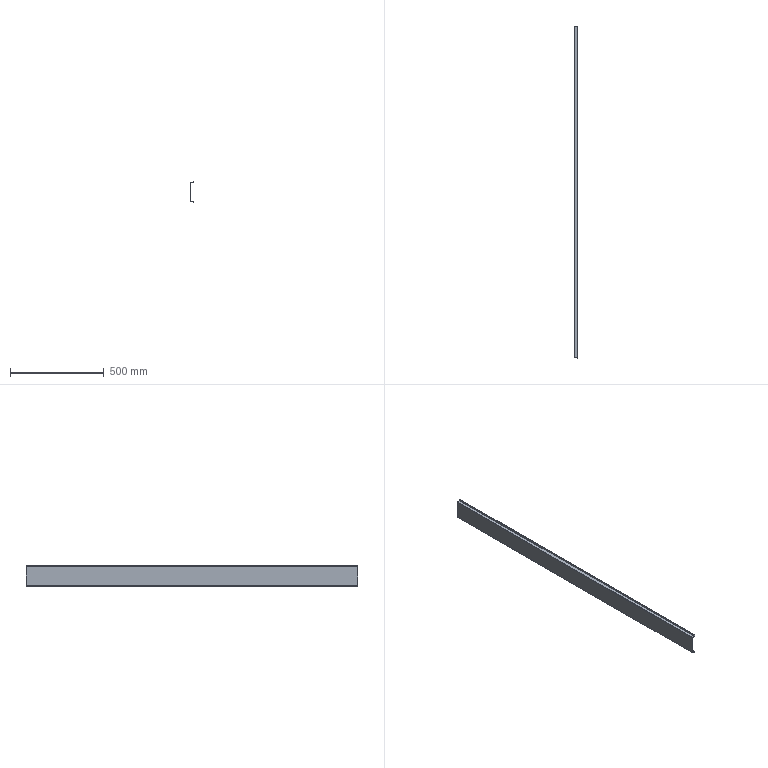Component | SolidWorks | RearDoorPanelWeldment-1_RearDoorStiffener-1 | 1 solid | 38 faces | box 18.9 x 1772 x 117 mm | volume 268936 mm3 | plane 30 | cylinder 8 | commonest cylinder face diameters 2.2 x4 0.2 x4
STEP:
#1=COLOUR_RGB('',0.7922,0.8196,0.9333);
#2=FILL_AREA_STYLE_COLOUR('',#1);
#3=FILL_AREA_STYLE('',(#2));
#4=SURFACE_STYLE_FILL_AREA(#3);
#5=SURFACE_SIDE_STYLE('',(#4));
#6=SURFACE_STYLE_USAGE(.BOTH.,#5);
#7=PRESENTATION_STYLE_ASSIGNMENT((#6));
#8=CARTESIAN_POINT('',(22.369,-36.828,72.855));
#9=VERTEX_POINT('',#8);
#10=CARTESIAN_POINT('',(23.027,-36.828,72.855));
#11=VERTEX_POINT('',#10);
#12=CARTESIAN_POINT('',(23.07,-36.828,72.855));
#13=DIRECTION('',(1.,0.,-0.));
#14=VECTOR('',#13,39.37);
#15=LINE('',#12,#14);
#16=EDGE_CURVE('',#9,#11,#15,.T.);
#17=ORIENTED_EDGE('',*,*,#16,.T.);
#18=CARTESIAN_POINT('',(23.027,-36.828,72.894));
#19=VERTEX_POINT('',#18);
#20=CARTESIAN_POINT('',(23.027,-36.828,72.855));
#21=DIRECTION('',(0.,0.,1.));
#22=VECTOR('',#21,39.37);
#23=LINE('',#20,#22);
#24=EDGE_CURVE('',#11,#19,#23,.T.);
#25=ORIENTED_EDGE('',*,*,#24,.T.);
#26=CARTESIAN_POINT('',(22.369,-36.828,72.894));
#27=VERTEX_POINT('',#26);
#28=CARTESIAN_POINT('',(22.326,-36.828,72.894));
#29=DIRECTION('',(1.,0.,-0.));
#30=VECTOR('',#29,39.37);
#31=LINE('',#28,#30);
#32=EDGE_CURVE('',#27,#19,#31,.T.);
#33=ORIENTED_EDGE('',*,*,#32,.F.);
#34=CARTESIAN_POINT('',(22.369,-36.828,72.855));
#35=DIRECTION('',(-0.,-0.,-1.));
#36=VECTOR('',#35,39.37);
#37=LINE('',#34,#36);
#38=EDGE_CURVE('',#27,#9,#37,.T.);
#39=ORIENTED_EDGE('',*,*,#38,.T.);
#40=EDGE_LOOP('',(#17,#25,#33,#39));
#41=FACE_OUTER_BOUND('',#40,.T.);
#42=CARTESIAN_POINT('',(23.07,-36.828,72.855));
#43=DIRECTION('',(0.,-1.,0.));
#44=DIRECTION('',(1.,0.,-0.));
#45=AXIS2_PLACEMENT_3D('',#42,#43,#44);
#46=PLANE('',#45);
#47=ADVANCED_FACE('',(#41),#46,.T.);
#48=CARTESIAN_POINT('',(23.027,32.936,72.855));
#49=VERTEX_POINT('',#48);
#50=CARTESIAN_POINT('',(22.369,32.936,72.855));
#51=VERTEX_POINT('',#50);
#52=CARTESIAN_POINT('',(22.365,32.936,72.855));
#53=DIRECTION('',(-1.,-0.,0.));
#54=VECTOR('',#53,39.37);
#55=LINE('',#52,#54);
#56=EDGE_CURVE('',#49,#51,#55,.T.);
#57=ORIENTED_EDGE('',*,*,#56,.F.);
#58=CARTESIAN_POINT('',(23.027,-36.828,72.855));
#59=DIRECTION('',(-0.,1.,-0.));
#60=VECTOR('',#59,39.37);
#61=LINE('',#58,#60);
#62=EDGE_CURVE('',#11,#49,#61,.T.);
#63=ORIENTED_EDGE('',*,*,#62,.F.);
#64=ORIENTED_EDGE('',*,*,#16,.F.);
#65=CARTESIAN_POINT('',(22.369,30.625,72.855));
#66=DIRECTION('',(-0.,1.,-0.));
#67=VECTOR('',#66,39.37);
#68=LINE('',#65,#67);
#69=EDGE_CURVE('',#9,#51,#68,.T.);
#70=ORIENTED_EDGE('',*,*,#69,.T.);
#71=EDGE_LOOP('',(#57,#63,#64,#70));
#72=FACE_OUTER_BOUND('',#71,.T.);
#73=CARTESIAN_POINT('',(22.326,30.625,72.855));
#74=DIRECTION('',(-0.,-0.,-1.));
#75=DIRECTION('',(1.,0.,-0.));
#76=AXIS2_PLACEMENT_3D('',#73,#74,#75);
#77=PLANE('',#76);
#78=ADVANCED_FACE('',(#72),#77,.T.);
#79=CARTESIAN_POINT('',(23.027,32.936,72.894));
#80=VERTEX_POINT('',#79);
#81=CARTESIAN_POINT('',(23.027,-36.828,72.894));
#82=DIRECTION('',(-0.,1.,-0.));
#83=VECTOR('',#82,39.37);
#84=LINE('',#81,#83);
#85=EDGE_CURVE('',#19,#80,#84,.T.);
#86=ORIENTED_EDGE('',*,*,#85,.T.);
#87=CARTESIAN_POINT('',(22.369,32.936,72.894));
#88=VERTEX_POINT('',#87);
#89=CARTESIAN_POINT('',(22.326,32.936,72.894));
#90=DIRECTION('',(-1.,-0.,0.));
#91=VECTOR('',#90,39.37);
#92=LINE('',#89,#91);
#93=EDGE_CURVE('',#80,#88,#92,.T.);
#94=ORIENTED_EDGE('',*,*,#93,.T.);
#95=CARTESIAN_POINT('',(22.369,-36.828,72.894));
#96=DIRECTION('',(-0.,1.,-0.));
#97=VECTOR('',#96,39.37);
#98=LINE('',#95,#97);
#99=EDGE_CURVE('',#27,#88,#98,.T.);
#100=ORIENTED_EDGE('',*,*,#99,.F.);
#101=ORIENTED_EDGE('',*,*,#32,.T.);
#102=EDGE_LOOP('',(#86,#94,#100,#101));
#103=FACE_OUTER_BOUND('',#102,.T.);
#104=CARTESIAN_POINT('',(22.326,30.625,72.894));
#105=DIRECTION('',(-0.,-0.,-1.));
#106=DIRECTION('',(1.,0.,-0.));
#107=AXIS2_PLACEMENT_3D('',#104,#105,#106);
#108=PLANE('',#107);
#109=ADVANCED_FACE('',(#103),#108,.F.);
#110=CARTESIAN_POINT('',(22.369,32.936,76.752));
#111=VERTEX_POINT('',#110);
#112=CARTESIAN_POINT('',(23.027,32.936,76.752));
#113=VERTEX_POINT('',#112);
#114=CARTESIAN_POINT('',(23.07,32.936,76.752));
#115=DIRECTION('',(1.,0.,-0.));
#116=VECTOR('',#115,39.37);
#117=LINE('',#114,#116);
#118=EDGE_CURVE('',#111,#113,#117,.T.);
#119=ORIENTED_EDGE('',*,*,#118,.T.);
#120=CARTESIAN_POINT('',(23.027,32.936,76.713));
#121=VERTEX_POINT('',#120);
#122=CARTESIAN_POINT('',(23.027,32.936,76.752));
#123=DIRECTION('',(-0.,-0.,-1.));
#124=VECTOR('',#123,39.37);
#125=LINE('',#122,#124);
#126=EDGE_CURVE('',#113,#121,#125,.T.);
#127=ORIENTED_EDGE('',*,*,#126,.T.);
#128=CARTESIAN_POINT('',(22.369,32.936,76.713));
#129=VERTEX_POINT('',#128);
#130=CARTESIAN_POINT('',(22.326,32.936,76.713));
#131=DIRECTION('',(1.,0.,-0.));
#132=VECTOR('',#131,39.37);
#133=LINE('',#130,#132);
#134=EDGE_CURVE('',#129,#121,#133,.T.);
#135=ORIENTED_EDGE('',*,*,#134,.F.);
#136=CARTESIAN_POINT('',(22.369,32.936,76.752));
#137=DIRECTION('',(0.,0.,1.));
#138=VECTOR('',#137,39.37);
#139=LINE('',#136,#138);
#140=EDGE_CURVE('',#129,#111,#139,.T.);
#141=ORIENTED_EDGE('',*,*,#140,.T.);
#142=EDGE_LOOP('',(#119,#127,#135,#141));
#143=FACE_OUTER_BOUND('',#142,.T.);
#144=CARTESIAN_POINT('',(23.07,32.936,76.752));
#145=DIRECTION('',(-0.,1.,-0.));
#146=DIRECTION('',(-1.,-0.,0.));
#147=AXIS2_PLACEMENT_3D('',#144,#145,#146);
#148=PLANE('',#147);
#149=ADVANCED_FACE('',(#143),#148,.T.);
#150=CARTESIAN_POINT('',(23.027,-36.828,76.752));
#151=VERTEX_POINT('',#150);
#152=CARTESIAN_POINT('',(22.369,-36.828,76.752));
#153=VERTEX_POINT('',#152);
#154=CARTESIAN_POINT('',(22.365,-36.828,76.752));
#155=DIRECTION('',(-1.,-0.,0.));
#156=VECTOR('',#155,39.37);
#157=LINE('',#154,#156);
#158=EDGE_CURVE('',#151,#153,#157,.T.);
#159=ORIENTED_EDGE('',*,*,#158,.F.);
#160=CARTESIAN_POINT('',(23.027,32.936,76.752));
#161=DIRECTION('',(0.,-1.,0.));
#162=VECTOR('',#161,39.37);
#163=LINE('',#160,#162);
#164=EDGE_CURVE('',#113,#151,#163,.T.);
#165=ORIENTED_EDGE('',*,*,#164,.F.);
#166=ORIENTED_EDGE('',*,*,#118,.F.);
#167=CARTESIAN_POINT('',(22.369,30.625,76.752));
#168=DIRECTION('',(0.,-1.,0.));
#169=VECTOR('',#168,39.37);
#170=LINE('',#167,#169);
#171=EDGE_CURVE('',#111,#153,#170,.T.);
#172=ORIENTED_EDGE('',*,*,#171,.T.);
#173=EDGE_LOOP('',(#159,#165,#166,#172));
#174=FACE_OUTER_BOUND('',#173,.T.);
#175=CARTESIAN_POINT('',(22.326,30.625,76.752));
#176=DIRECTION('',(0.,0.,1.));
#177=DIRECTION('',(-1.,-0.,0.));
#178=AXIS2_PLACEMENT_3D('',#175,#176,#177);
#179=PLANE('',#178);
#180=ADVANCED_FACE('',(#174),#179,.T.);
#181=CARTESIAN_POINT('',(23.027,-36.828,76.713));
#182=VERTEX_POINT('',#181);
#183=CARTESIAN_POINT('',(23.027,32.936,76.713));
#184=DIRECTION('',(0.,-1.,0.));
#185=VECTOR('',#184,39.37);
#186=LINE('',#183,#185);
#187=EDGE_CURVE('',#121,#182,#186,.T.);
#188=ORIENTED_EDGE('',*,*,#187,.T.);
#189=CARTESIAN_POINT('',(22.369,-36.828,76.713));
#190=VERTEX_POINT('',#189);
#191=CARTESIAN_POINT('',(22.326,-36.828,76.713));
#192=DIRECTION('',(-1.,-0.,0.));
#193=VECTOR('',#192,39.37);
#194=LINE('',#191,#193);
#195=EDGE_CURVE('',#182,#190,#194,.T.);
#196=ORIENTED_EDGE('',*,*,#195,.T.);
#197=CARTESIAN_POINT('',(22.369,32.936,76.713));
#198=DIRECTION('',(0.,-1.,0.));
#199=VECTOR('',#198,39.37);
#200=LINE('',#197,#199);
#201=EDGE_CURVE('',#129,#190,#200,.T.);
#202=ORIENTED_EDGE('',*,*,#201,.F.);
#203=ORIENTED_EDGE('',*,*,#134,.T.);
#204=EDGE_LOOP('',(#188,#196,#202,#203));
#205=FACE_OUTER_BOUND('',#204,.T.);
#206=CARTESIAN_POINT('',(22.326,30.625,76.713));
#207=DIRECTION('',(0.,0.,1.));
#208=DIRECTION('',(-1.,-0.,0.));
#209=AXIS2_PLACEMENT_3D('',#206,#207,#208);
#210=PLANE('',#209);
#211=ADVANCED_FACE('',(#205),#210,.F.);
#212=CARTESIAN_POINT('',(22.365,32.936,72.898));
#213=VERTEX_POINT('',#212);
#214=CARTESIAN_POINT('',(22.365,-36.828,72.898));
#215=VERTEX_POINT('',#214);
#216=CARTESIAN_POINT('',(22.365,32.936,72.898));
#217=DIRECTION('',(0.,-1.,0.));
#218=VECTOR('',#217,39.37);
#219=LINE('',#216,#218);
#220=EDGE_CURVE('',#213,#215,#219,.T.);
#221=ORIENTED_EDGE('',*,*,#220,.F.);
#222=CARTESIAN_POINT('',(22.365,32.936,76.709));
#223=VERTEX_POINT('',#222);
#224=CARTESIAN_POINT('',(22.365,32.936,76.752));
#225=DIRECTION('',(-0.,-0.,-1.));
#226=VECTOR('',#225,39.37);
#227=LINE('',#224,#226);
#228=EDGE_CURVE('',#223,#213,#227,.T.);
#229=ORIENTED_EDGE('',*,*,#228,.F.);
#230=CARTESIAN_POINT('',(22.365,-36.828,76.709));
#231=VERTEX_POINT('',#230);
#232=CARTESIAN_POINT('',(22.365,-36.828,76.709));
#233=DIRECTION('',(-0.,1.,-0.));
#234=VECTOR('',#233,39.37);
#235=LINE('',#232,#234);
#236=EDGE_CURVE('',#231,#223,#235,.T.);
#237=ORIENTED_EDGE('',*,*,#236,.F.);
#238=CARTESIAN_POINT('',(22.365,-36.828,76.752));
#239=DIRECTION('',(0.,0.,1.));
#240=VECTOR('',#239,39.37);
#241=LINE('',#238,#240);
#242=EDGE_CURVE('',#215,#231,#241,.T.);
#243=ORIENTED_EDGE('',*,*,#242,.F.);
#244=EDGE_LOOP('',(#221,#229,#237,#243));
#245=FACE_OUTER_BOUND('',#244,.T.);
#246=CARTESIAN_POINT('',(22.365,30.625,74.593));
#247=DIRECTION('',(-1.,-0.,0.));
#248=DIRECTION('',(0.,-1.,0.));
#249=AXIS2_PLACEMENT_3D('',#246,#247,#248);
#250=PLANE('',#249);
#251=ADVANCED_FACE('',(#245),#250,.F.);
#252=CARTESIAN_POINT('',(22.326,32.936,76.709));
#253=VERTEX_POINT('',#252);
#254=CARTESIAN_POINT('',(22.326,32.936,72.898));
#255=VERTEX_POINT('',#254);
#256=CARTESIAN_POINT('',(22.326,32.936,76.752));
#257=DIRECTION('',(-0.,-0.,-1.));
#258=VECTOR('',#257,39.37);
#259=LINE('',#256,#258);
#260=EDGE_CURVE('',#253,#255,#259,.T.);
#261=ORIENTED_EDGE('',*,*,#260,.T.);
#262=CARTESIAN_POINT('',(22.326,-36.828,72.898));
#263=VERTEX_POINT('',#262);
#264=CARTESIAN_POINT('',(22.326,32.936,72.898));
#265=DIRECTION('',(0.,-1.,0.));
#266=VECTOR('',#265,39.37);
#267=LINE('',#264,#266);
#268=EDGE_CURVE('',#255,#263,#267,.T.);
#269=ORIENTED_EDGE('',*,*,#268,.T.);
#270=CARTESIAN_POINT('',(22.326,-36.828,76.709));
#271=VERTEX_POINT('',#270);
#272=CARTESIAN_POINT('',(22.326,-36.828,76.752));
#273=DIRECTION('',(0.,0.,1.));
#274=VECTOR('',#273,39.37);
#275=LINE('',#272,#274);
#276=EDGE_CURVE('',#263,#271,#275,.T.);
#277=ORIENTED_EDGE('',*,*,#276,.T.);
#278=CARTESIAN_POINT('',(22.326,-36.828,76.709));
#279=DIRECTION('',(-0.,1.,-0.));
#280=VECTOR('',#279,39.37);
#281=LINE('',#278,#280);
#282=EDGE_CURVE('',#271,#253,#281,.T.);
#283=ORIENTED_EDGE('',*,*,#282,.T.);
#284=EDGE_LOOP('',(#261,#269,#277,#283));
#285=FACE_OUTER_BOUND('',#284,.T.);
#286=CARTESIAN_POINT('',(22.326,30.625,74.593));
#287=DIRECTION('',(-1.,-0.,0.));
#288=DIRECTION('',(0.,-1.,0.));
#289=AXIS2_PLACEMENT_3D('',#286,#287,#288);
#290=PLANE('',#289);
#291=ADVANCED_FACE('',(#285),#290,.T.);
#292=ORIENTED_EDGE('',*,*,#228,.T.);
#293=CARTESIAN_POINT('',(22.365,32.936,72.898));
#294=DIRECTION('',(-1.,-0.,0.));
#295=VECTOR('',#294,39.37);
#296=LINE('',#293,#295);
#297=EDGE_CURVE('',#213,#255,#296,.T.);
#298=ORIENTED_EDGE('',*,*,#297,.T.);
#299=ORIENTED_EDGE('',*,*,#260,.F.);
#300=CARTESIAN_POINT('',(22.365,32.936,76.709));
#301=DIRECTION('',(-1.,0.,0.));
#302=VECTOR('',#301,39.37);
#303=LINE('',#300,#302);
#304=EDGE_CURVE('',#223,#253,#303,.T.);
#305=ORIENTED_EDGE('',*,*,#304,.F.);
#306=EDGE_LOOP('',(#292,#298,#299,#305));
#307=FACE_OUTER_BOUND('',#306,.T.);
#308=CARTESIAN_POINT('',(22.365,32.936,76.752));
#309=DIRECTION('',(-0.,1.,-0.));
#310=DIRECTION('',(-0.,-0.,-1.));
#311=AXIS2_PLACEMENT_3D('',#308,#309,#310);
#312=PLANE('',#311);
#313=ADVANCED_FACE('',(#307),#312,.T.);
#314=CARTESIAN_POINT('',(22.365,-36.828,72.898));
#315=DIRECTION('',(-1.,-0.,0.));
#316=VECTOR('',#315,39.37);
#317=LINE('',#314,#316);
#318=EDGE_CURVE('',#215,#263,#317,.T.);
#319=ORIENTED_EDGE('',*,*,#318,.F.);
#320=ORIENTED_EDGE('',*,*,#242,.T.);
#321=CARTESIAN_POINT('',(22.365,-36.828,76.709));
#322=DIRECTION('',(-1.,-0.,0.));
#323=VECTOR('',#322,39.37);
#324=LINE('',#321,#323);
#325=EDGE_CURVE('',#231,#271,#324,.T.);
#326=ORIENTED_EDGE('',*,*,#325,.T.);
#327=ORIENTED_EDGE('',*,*,#276,.F.);
#328=EDGE_LOOP('',(#319,#320,#326,#327));
#329=FACE_OUTER_BOUND('',#328,.T.);
#330=CARTESIAN_POINT('',(22.365,-36.828,76.752));
#331=DIRECTION('',(0.,-1.,0.));
#332=DIRECTION('',(1.,0.,-0.));
#333=AXIS2_PLACEMENT_3D('',#330,#331,#332);
#334=PLANE('',#333);
#335=ADVANCED_FACE('',(#329),#334,.T.);
#336=ORIENTED_EDGE('',*,*,#140,.F.);
#337=CARTESIAN_POINT('',(22.369,32.936,76.709));
#338=DIRECTION('',(-0.,1.,-0.));
#339=DIRECTION('',(1.,0.,0.));
#340=AXIS2_PLACEMENT_3D('',#337,#338,#339);
#341=CIRCLE('',#340,0.003937);
#342=EDGE_CURVE('',#223,#129,#341,.T.);
#343=ORIENTED_EDGE('',*,*,#342,.F.);
#344=ORIENTED_EDGE('',*,*,#304,.T.);
#345=CARTESIAN_POINT('',(22.369,32.936,76.709));
#346=DIRECTION('',(-0.,1.,-0.));
#347=DIRECTION('',(1.,0.,0.));
#348=AXIS2_PLACEMENT_3D('',#345,#346,#347);
#349=CIRCLE('',#348,0.04331);
#350=EDGE_CURVE('',#253,#111,#349,.T.);
#351=ORIENTED_EDGE('',*,*,#350,.T.);
#352=EDGE_LOOP('',(#336,#343,#344,#351));
#353=FACE_OUTER_BOUND('',#352,.T.);
#354=CARTESIAN_POINT('',(22.369,32.936,76.709));
#355=DIRECTION('',(-0.,1.,-0.));
#356=DIRECTION('',(-1.,-0.,0.));
#357=AXIS2_PLACEMENT_3D('',#354,#355,#356);
#358=PLANE('',#357);
#359=ADVANCED_FACE('',(#353),#358,.T.);
#360=CARTESIAN_POINT('',(22.369,-36.828,76.709));
#361=DIRECTION('',(0.,-1.,0.));
#362=DIRECTION('',(1.,0.,0.));
#363=AXIS2_PLACEMENT_3D('',#360,#361,#362);
#364=CIRCLE('',#363,0.003937);
#365=EDGE_CURVE('',#190,#231,#364,.T.);
#366=ORIENTED_EDGE('',*,*,#365,.F.);
#367=CARTESIAN_POINT('',(22.369,-36.828,76.713));
#368=DIRECTION('',(0.,0.,1.));
#369=VECTOR('',#368,39.37);
#370=LINE('',#367,#369);
#371=EDGE_CURVE('',#190,#153,#370,.T.);
#372=ORIENTED_EDGE('',*,*,#371,.T.);
#373=CARTESIAN_POINT('',(22.369,-36.828,76.709));
#374=DIRECTION('',(0.,-1.,0.));
#375=DIRECTION('',(1.,0.,0.));
#376=AXIS2_PLACEMENT_3D('',#373,#374,#375);
#377=CIRCLE('',#376,0.04331);
#378=EDGE_CURVE('',#153,#271,#377,.T.);
#379=ORIENTED_EDGE('',*,*,#378,.T.);
#380=ORIENTED_EDGE('',*,*,#325,.F.);
#381=EDGE_LOOP('',(#366,#372,#379,#380));
#382=FACE_OUTER_BOUND('',#381,.T.);
#383=CARTESIAN_POINT('',(22.369,-36.828,76.709));
#384=DIRECTION('',(-0.,1.,-0.));
#385=DIRECTION('',(-1.,-0.,0.));
#386=AXIS2_PLACEMENT_3D('',#383,#384,#385);
#387=PLANE('',#386);
#388=ADVANCED_FACE('',(#382),#387,.F.);
#389=ORIENTED_EDGE('',*,*,#282,.F.);
#390=ORIENTED_EDGE('',*,*,#378,.F.);
#391=ORIENTED_EDGE('',*,*,#171,.F.);
#392=ORIENTED_EDGE('',*,*,#350,.F.);
#393=EDGE_LOOP('',(#389,#390,#391,#392));
#394=FACE_OUTER_BOUND('',#393,.T.);
#395=CARTESIAN_POINT('',(22.369,-36.828,76.709));
#396=DIRECTION('',(0.,-1.,0.));
#397=DIRECTION('',(0.,0.,1.));
#398=AXIS2_PLACEMENT_3D('',#395,#396,#397);
#399=CYLINDRICAL_SURFACE('',#398,0.04331);
#400=ADVANCED_FACE('',(#394),#399,.T.);
#401=ORIENTED_EDGE('',*,*,#236,.T.);
#402=ORIENTED_EDGE('',*,*,#342,.T.);
#403=ORIENTED_EDGE('',*,*,#201,.T.);
#404=ORIENTED_EDGE('',*,*,#365,.T.);
#405=EDGE_LOOP('',(#401,#402,#403,#404));
#406=FACE_OUTER_BOUND('',#405,.T.);
#407=CARTESIAN_POINT('',(22.369,-36.828,76.709));
#408=DIRECTION('',(0.,-1.,0.));
#409=DIRECTION('',(0.,0.,1.));
#410=AXIS2_PLACEMENT_3D('',#407,#408,#409);
#411=CYLINDRICAL_SURFACE('',#410,0.003937);
#412=ADVANCED_FACE('',(#406),#411,.F.);
#413=CARTESIAN_POINT('',(23.027,-36.828,76.752));
#414=DIRECTION('',(-0.,-0.,-1.));
#415=VECTOR('',#414,39.37);
#416=LINE('',#413,#415);
#417=EDGE_CURVE('',#151,#182,#416,.T.);
#418=ORIENTED_EDGE('',*,*,#417,.F.);
#419=ORIENTED_EDGE('',*,*,#158,.T.);
#420=ORIENTED_EDGE('',*,*,#371,.F.);
#421=ORIENTED_EDGE('',*,*,#195,.F.);
#422=EDGE_LOOP('',(#418,#419,#420,#421));
#423=FACE_OUTER_BOUND('',#422,.T.);
#424=CARTESIAN_POINT('',(22.365,-36.828,76.752));
#425=DIRECTION('',(0.,-1.,0.));
#426=DIRECTION('',(1.,0.,-0.));
#427=AXIS2_PLACEMENT_3D('',#424,#425,#426);
#428=PLANE('',#427);
#429=ADVANCED_FACE('',(#423),#428,.T.);
#430=ORIENTED_EDGE('',*,*,#38,.F.);
#431=CARTESIAN_POINT('',(22.369,-36.828,72.898));
#432=DIRECTION('',(0.,-1.,0.));
#433=DIRECTION('',(-1.,0.,0.));
#434=AXIS2_PLACEMENT_3D('',#431,#432,#433);
#435=CIRCLE('',#434,0.003937);
#436=EDGE_CURVE('',#215,#27,#435,.T.);
#437=ORIENTED_EDGE('',*,*,#436,.F.);
#438=ORIENTED_EDGE('',*,*,#318,.T.);
#439=CARTESIAN_POINT('',(22.369,-36.828,72.898));
#440=DIRECTION('',(0.,-1.,0.));
#441=DIRECTION('',(-1.,0.,0.));
#442=AXIS2_PLACEMENT_3D('',#439,#440,#441);
#443=CIRCLE('',#442,0.04331);
#444=EDGE_CURVE('',#263,#9,#443,.T.);
#445=ORIENTED_EDGE('',*,*,#444,.T.);
#446=EDGE_LOOP('',(#430,#437,#438,#445));
#447=FACE_OUTER_BOUND('',#446,.T.);
#448=CARTESIAN_POINT('',(22.369,-36.828,72.898));
#449=DIRECTION('',(0.,-1.,0.));
#450=DIRECTION('',(1.,0.,-0.));
#451=AXIS2_PLACEMENT_3D('',#448,#449,#450);
#452=PLANE('',#451);
#453=ADVANCED_FACE('',(#447),#452,.T.);
#454=CARTESIAN_POINT('',(22.369,32.936,72.898));
#455=DIRECTION('',(-0.,1.,-0.));
#456=DIRECTION('',(-1.,0.,0.));
#457=AXIS2_PLACEMENT_3D('',#454,#455,#456);
#458=CIRCLE('',#457,0.003937);
#459=EDGE_CURVE('',#88,#213,#458,.T.);
#460=ORIENTED_EDGE('',*,*,#459,.F.);
#461=CARTESIAN_POINT('',(22.369,32.936,72.894));
#462=DIRECTION('',(-0.,-0.,-1.));
#463=VECTOR('',#462,39.37);
#464=LINE('',#461,#463);
#465=EDGE_CURVE('',#88,#51,#464,.T.);
#466=ORIENTED_EDGE('',*,*,#465,.T.);
#467=CARTESIAN_POINT('',(22.369,32.936,72.898));
#468=DIRECTION('',(-0.,1.,-0.));
#469=DIRECTION('',(-1.,0.,0.));
#470=AXIS2_PLACEMENT_3D('',#467,#468,#469);
#471=CIRCLE('',#470,0.04331);
#472=EDGE_CURVE('',#51,#255,#471,.T.);
#473=ORIENTED_EDGE('',*,*,#472,.T.);
#474=ORIENTED_EDGE('',*,*,#297,.F.);
#475=EDGE_LOOP('',(#460,#466,#473,#474));
#476=FACE_OUTER_BOUND('',#475,.T.);
#477=CARTESIAN_POINT('',(22.369,32.936,72.898));
#478=DIRECTION('',(0.,-1.,0.));
#479=DIRECTION('',(1.,0.,-0.));
#480=AXIS2_PLACEMENT_3D('',#477,#478,#479);
#481=PLANE('',#480);
#482=ADVANCED_FACE('',(#476),#481,.F.);
#483=ORIENTED_EDGE('',*,*,#268,.F.);
#484=ORIENTED_EDGE('',*,*,#472,.F.);
#485=ORIENTED_EDGE('',*,*,#69,.F.);
#486=ORIENTED_EDGE('',*,*,#444,.F.);
#487=EDGE_LOOP('',(#483,#484,#485,#486));
#488=FACE_OUTER_BOUND('',#487,.T.);
#489=CARTESIAN_POINT('',(22.369,32.936,72.898));
#490=DIRECTION('',(-0.,1.,-0.));
#491=DIRECTION('',(0.,0.,-1.));
#492=AXIS2_PLACEMENT_3D('',#489,#490,#491);
#493=CYLINDRICAL_SURFACE('',#492,0.04331);
#494=ADVANCED_FACE('',(#488),#493,.T.);
#495=ORIENTED_EDGE('',*,*,#220,.T.);
#496=ORIENTED_EDGE('',*,*,#436,.T.);
#497=ORIENTED_EDGE('',*,*,#99,.T.);
#498=ORIENTED_EDGE('',*,*,#459,.T.);
#499=EDGE_LOOP('',(#495,#496,#497,#498));
#500=FACE_OUTER_BOUND('',#499,.T.);
#501=CARTESIAN_POINT('',(22.369,32.936,72.898));
#502=DIRECTION('',(-0.,1.,-0.));
#503=DIRECTION('',(0.,0.,-1.));
#504=AXIS2_PLACEMENT_3D('',#501,#502,#503);
#505=CYLINDRICAL_SURFACE('',#504,0.003937);
#506=ADVANCED_FACE('',(#500),#505,.F.);
#507=CARTESIAN_POINT('',(23.027,32.936,72.855));
#508=DIRECTION('',(0.,0.,1.));
#509=VECTOR('',#508,39.37);
#510=LINE('',#507,#509);
#511=EDGE_CURVE('',#49,#80,#510,.T.);
#512=ORIENTED_EDGE('',*,*,#511,.F.);
#513=ORIENTED_EDGE('',*,*,#56,.T.);
#514=ORIENTED_EDGE('',*,*,#465,.F.);
#515=ORIENTED_EDGE('',*,*,#93,.F.);
#516=EDGE_LOOP('',(#512,#513,#514,#515));
#517=FACE_OUTER_BOUND('',#516,.T.);
#518=CARTESIAN_POINT('',(22.365,32.936,72.855));
#519=DIRECTION('',(-0.,1.,-0.));
#520=DIRECTION('',(-1.,-0.,0.));
#521=AXIS2_PLACEMENT_3D('',#518,#519,#520);
#522=PLANE('',#521);
#523=ADVANCED_FACE('',(#517),#522,.T.);
#524=CARTESIAN_POINT('',(23.031,-36.828,76.756));
#525=VERTEX_POINT('',#524);
#526=CARTESIAN_POINT('',(23.07,-36.828,76.756));
#527=VERTEX_POINT('',#526);
#528=CARTESIAN_POINT('',(23.07,-36.828,76.756));
#529=DIRECTION('',(1.,0.,0.));
#530=VECTOR('',#529,39.37);
#531=LINE('',#528,#530);
#532=EDGE_CURVE('',#525,#527,#531,.T.);
#533=ORIENTED_EDGE('',*,*,#532,.F.);
#534=CARTESIAN_POINT('',(23.027,-36.828,76.756));
#535=DIRECTION('',(0.,-1.,0.));
#536=DIRECTION('',(-1.,0.,0.));
#537=AXIS2_PLACEMENT_3D('',#534,#535,#536);
#538=CIRCLE('',#537,0.003937);
#539=EDGE_CURVE('',#151,#525,#538,.T.);
#540=ORIENTED_EDGE('',*,*,#539,.F.);
#541=ORIENTED_EDGE('',*,*,#417,.T.);
#542=CARTESIAN_POINT('',(23.027,-36.828,76.756));
#543=DIRECTION('',(0.,-1.,0.));
#544=DIRECTION('',(-1.,0.,0.));
#545=AXIS2_PLACEMENT_3D('',#542,#543,#544);
#546=CIRCLE('',#545,0.04331);
#547=EDGE_CURVE('',#182,#527,#546,.T.);
#548=ORIENTED_EDGE('',*,*,#547,.T.);
#549=EDGE_LOOP('',(#533,#540,#541,#548));
#550=FACE_OUTER_BOUND('',#549,.T.);
#551=CARTESIAN_POINT('',(23.027,-36.828,76.756));
#552=DIRECTION('',(0.,-1.,0.));
#553=DIRECTION('',(1.,0.,-0.));
#554=AXIS2_PLACEMENT_3D('',#551,#552,#553);
#555=PLANE('',#554);
#556=ADVANCED_FACE('',(#550),#555,.T.);
#557=CARTESIAN_POINT('',(23.031,32.936,76.756));
#558=VERTEX_POINT('',#557);
#559=CARTESIAN_POINT('',(23.027,32.936,76.756));
#560=DIRECTION('',(-0.,1.,-0.));
#561=DIRECTION('',(-1.,0.,0.));
#562=AXIS2_PLACEMENT_3D('',#559,#560,#561);
#563=CIRCLE('',#562,0.003937);
#564=EDGE_CURVE('',#558,#113,#563,.T.);
#565=ORIENTED_EDGE('',*,*,#564,.F.);
#566=CARTESIAN_POINT('',(23.07,32.936,76.756));
#567=VERTEX_POINT('',#566);
#568=CARTESIAN_POINT('',(23.031,32.936,76.756));
#569=DIRECTION('',(1.,0.,0.));
#570=VECTOR('',#569,39.37);
#571=LINE('',#568,#570);
#572=EDGE_CURVE('',#558,#567,#571,.T.);
#573=ORIENTED_EDGE('',*,*,#572,.T.);
#574=CARTESIAN_POINT('',(23.027,32.936,76.756));
#575=DIRECTION('',(-0.,1.,-0.));
#576=DIRECTION('',(-1.,0.,0.));
#577=AXIS2_PLACEMENT_3D('',#574,#575,#576);
#578=CIRCLE('',#577,0.04331);
#579=EDGE_CURVE('',#567,#121,#578,.T.);
#580=ORIENTED_EDGE('',*,*,#579,.T.);
#581=ORIENTED_EDGE('',*,*,#126,.F.);
#582=EDGE_LOOP('',(#565,#573,#580,#581));
#583=FACE_OUTER_BOUND('',#582,.T.);
#584=CARTESIAN_POINT('',(23.027,32.936,76.756));
#585=DIRECTION('',(0.,-1.,0.));
#586=DIRECTION('',(1.,0.,-0.));
#587=AXIS2_PLACEMENT_3D('',#584,#585,#586);
#588=PLANE('',#587);
#589=ADVANCED_FACE('',(#583),#588,.F.);
#590=ORIENTED_EDGE('',*,*,#187,.F.);
#591=ORIENTED_EDGE('',*,*,#579,.F.);
#592=CARTESIAN_POINT('',(23.07,30.625,76.756));
#593=DIRECTION('',(-0.,1.,-0.));
#594=VECTOR('',#593,39.37);
#595=LINE('',#592,#594);
#596=EDGE_CURVE('',#527,#567,#595,.T.);
#597=ORIENTED_EDGE('',*,*,#596,.F.);
#598=ORIENTED_EDGE('',*,*,#547,.F.);
#599=EDGE_LOOP('',(#590,#591,#597,#598));
#600=FACE_OUTER_BOUND('',#599,.T.);
#601=CARTESIAN_POINT('',(23.027,32.936,76.756));
#602=DIRECTION('',(-0.,1.,-0.));
#603=DIRECTION('',(1.,0.,0.));
#604=AXIS2_PLACEMENT_3D('',#601,#602,#603);
#605=CYLINDRICAL_SURFACE('',#604,0.04331);
#606=ADVANCED_FACE('',(#600),#605,.T.);
#607=ORIENTED_EDGE('',*,*,#164,.T.);
#608=ORIENTED_EDGE('',*,*,#539,.T.);
#609=CARTESIAN_POINT('',(23.031,-36.828,76.756));
#610=DIRECTION('',(-0.,1.,-0.));
#611=VECTOR('',#610,39.37);
#612=LINE('',#609,#611);
#613=EDGE_CURVE('',#525,#558,#612,.T.);
#614=ORIENTED_EDGE('',*,*,#613,.T.);
#615=ORIENTED_EDGE('',*,*,#564,.T.);
#616=EDGE_LOOP('',(#607,#608,#614,#615));
#617=FACE_OUTER_BOUND('',#616,.T.);
#618=CARTESIAN_POINT('',(23.027,32.936,76.756));
#619=DIRECTION('',(-0.,1.,-0.));
#620=DIRECTION('',(1.,0.,0.));
#621=AXIS2_PLACEMENT_3D('',#618,#619,#620);
#622=CYLINDRICAL_SURFACE('',#621,0.003937);
#623=ADVANCED_FACE('',(#617),#622,.F.);
#624=CARTESIAN_POINT('',(23.07,32.936,77.107));
#625=VERTEX_POINT('',#624);
#626=CARTESIAN_POINT('',(23.07,32.936,76.752));
#627=DIRECTION('',(-0.,-0.,-1.));
#628=VECTOR('',#627,39.37);
#629=LINE('',#626,#628);
#630=EDGE_CURVE('',#625,#567,#629,.T.);
#631=ORIENTED_EDGE('',*,*,#630,.T.);
#632=ORIENTED_EDGE('',*,*,#572,.F.);
#633=CARTESIAN_POINT('',(23.031,32.936,77.107));
#634=VERTEX_POINT('',#633);
#635=CARTESIAN_POINT('',(23.031,32.936,74.593));
#636=DIRECTION('',(-0.,-0.,-1.));
#637=VECTOR('',#636,39.37);
#638=LINE('',#635,#637);
#639=EDGE_CURVE('',#634,#558,#638,.T.);
#640=ORIENTED_EDGE('',*,*,#639,.F.);
#641=CARTESIAN_POINT('',(23.07,32.936,77.107));
#642=DIRECTION('',(-1.,-0.,0.));
#643=VECTOR('',#642,39.37);
#644=LINE('',#641,#643);
#645=EDGE_CURVE('',#625,#634,#644,.T.);
#646=ORIENTED_EDGE('',*,*,#645,.F.);
#647=EDGE_LOOP('',(#631,#632,#640,#646));
#648=FACE_OUTER_BOUND('',#647,.T.);
#649=CARTESIAN_POINT('',(23.07,32.936,76.752));
#650=DIRECTION('',(-0.,1.,-0.));
#651=DIRECTION('',(-0.,-0.,-1.));
#652=AXIS2_PLACEMENT_3D('',#649,#650,#651);
#653=PLANE('',#652);
#654=ADVANCED_FACE('',(#648),#653,.T.);
#655=CARTESIAN_POINT('',(23.031,-36.828,77.107));
#656=VERTEX_POINT('',#655);
#657=CARTESIAN_POINT('',(23.031,-36.828,74.593));
#658=DIRECTION('',(0.,0.,1.));
#659=VECTOR('',#658,39.37);
#660=LINE('',#657,#659);
#661=EDGE_CURVE('',#525,#656,#660,.T.);
#662=ORIENTED_EDGE('',*,*,#661,.F.);
#663=ORIENTED_EDGE('',*,*,#532,.T.);
#664=CARTESIAN_POINT('',(23.07,-36.828,77.107));
#665=VERTEX_POINT('',#664);
#666=CARTESIAN_POINT('',(23.07,-36.828,77.107));
#667=DIRECTION('',(0.,0.,1.));
#668=VECTOR('',#667,39.37);
#669=LINE('',#666,#668);
#670=EDGE_CURVE('',#527,#665,#669,.T.);
#671=ORIENTED_EDGE('',*,*,#670,.T.);
#672=CARTESIAN_POINT('',(23.07,-36.828,77.107));
#673=DIRECTION('',(-1.,-0.,0.));
#674=VECTOR('',#673,39.37);
#675=LINE('',#672,#674);
#676=EDGE_CURVE('',#665,#656,#675,.T.);
#677=ORIENTED_EDGE('',*,*,#676,.T.);
#678=EDGE_LOOP('',(#662,#663,#671,#677));
#679=FACE_OUTER_BOUND('',#678,.T.);
#680=CARTESIAN_POINT('',(23.07,-36.828,77.107));
#681=DIRECTION('',(0.,-1.,0.));
#682=DIRECTION('',(1.,0.,-0.));
#683=AXIS2_PLACEMENT_3D('',#680,#681,#682);
#684=PLANE('',#683);
#685=ADVANCED_FACE('',(#679),#684,.T.);
#686=ORIENTED_EDGE('',*,*,#670,.F.);
#687=ORIENTED_EDGE('',*,*,#596,.T.);
#688=ORIENTED_EDGE('',*,*,#630,.F.);
#689=CARTESIAN_POINT('',(23.07,32.936,77.107));
#690=DIRECTION('',(-0.,1.,-0.));
#691=VECTOR('',#690,39.37);
#692=LINE('',#689,#691);
#693=EDGE_CURVE('',#665,#625,#692,.T.);
#694=ORIENTED_EDGE('',*,*,#693,.F.);
#695=EDGE_LOOP('',(#686,#687,#688,#694));
#696=FACE_OUTER_BOUND('',#695,.T.);
#697=CARTESIAN_POINT('',(23.07,30.625,74.593));
#698=DIRECTION('',(1.,0.,-0.));
#699=DIRECTION('',(-0.,1.,-0.));
#700=AXIS2_PLACEMENT_3D('',#697,#698,#699);
#701=PLANE('',#700);
#702=ADVANCED_FACE('',(#696),#701,.T.);
#703=ORIENTED_EDGE('',*,*,#613,.F.);
#704=ORIENTED_EDGE('',*,*,#661,.T.);
#705=CARTESIAN_POINT('',(23.031,30.625,77.107));
#706=DIRECTION('',(-0.,1.,-0.));
#707=VECTOR('',#706,39.37);
#708=LINE('',#705,#707);
#709=EDGE_CURVE('',#656,#634,#708,.T.);
#710=ORIENTED_EDGE('',*,*,#709,.T.);
#711=ORIENTED_EDGE('',*,*,#639,.T.);
#712=EDGE_LOOP('',(#703,#704,#710,#711));
#713=FACE_OUTER_BOUND('',#712,.T.);
#714=CARTESIAN_POINT('',(23.031,30.625,74.593));
#715=DIRECTION('',(1.,0.,-0.));
#716=DIRECTION('',(-0.,1.,-0.));
#717=AXIS2_PLACEMENT_3D('',#714,#715,#716);
#718=PLANE('',#717);
#719=ADVANCED_FACE('',(#713),#718,.F.);
#720=ORIENTED_EDGE('',*,*,#709,.F.);
#721=ORIENTED_EDGE('',*,*,#676,.F.);
#722=ORIENTED_EDGE('',*,*,#693,.T.);
#723=ORIENTED_EDGE('',*,*,#645,.T.);
#724=EDGE_LOOP('',(#720,#721,#722,#723));
#725=FACE_OUTER_BOUND('',#724,.T.);
#726=CARTESIAN_POINT('',(23.07,32.936,77.107));
#727=DIRECTION('',(0.,0.,1.));
#728=DIRECTION('',(-1.,-0.,0.));
#729=AXIS2_PLACEMENT_3D('',#726,#727,#728);
#730=PLANE('',#729);
#731=ADVANCED_FACE('',(#725),#730,.T.);
#732=CARTESIAN_POINT('',(23.031,32.936,72.851));
#733=VERTEX_POINT('',#732);
#734=CARTESIAN_POINT('',(23.07,32.936,72.851));
#735=VERTEX_POINT('',#734);
#736=CARTESIAN_POINT('',(23.07,32.936,72.851));
#737=DIRECTION('',(1.,0.,0.));
#738=VECTOR('',#737,39.37);
#739=LINE('',#736,#738);
#740=EDGE_CURVE('',#733,#735,#739,.T.);
#741=ORIENTED_EDGE('',*,*,#740,.F.);
#742=CARTESIAN_POINT('',(23.027,32.936,72.851));
#743=DIRECTION('',(-0.,1.,-0.));
#744=DIRECTION('',(1.,0.,0.));
#745=AXIS2_PLACEMENT_3D('',#742,#743,#744);
#746=CIRCLE('',#745,0.003937);
#747=EDGE_CURVE('',#49,#733,#746,.T.);
#748=ORIENTED_EDGE('',*,*,#747,.F.);
#749=ORIENTED_EDGE('',*,*,#511,.T.);
#750=CARTESIAN_POINT('',(23.027,32.936,72.851));
#751=DIRECTION('',(-0.,1.,-0.));
#752=DIRECTION('',(1.,0.,0.));
#753=AXIS2_PLACEMENT_3D('',#750,#751,#752);
#754=CIRCLE('',#753,0.04331);
#755=EDGE_CURVE('',#80,#735,#754,.T.);
#756=ORIENTED_EDGE('',*,*,#755,.T.);
#757=EDGE_LOOP('',(#741,#748,#749,#756));
#758=FACE_OUTER_BOUND('',#757,.T.);
#759=CARTESIAN_POINT('',(23.027,32.936,72.851));
#760=DIRECTION('',(-0.,1.,-0.));
#761=DIRECTION('',(-1.,-0.,0.));
#762=AXIS2_PLACEMENT_3D('',#759,#760,#761);
#763=PLANE('',#762);
#764=ADVANCED_FACE('',(#758),#763,.T.);
#765=CARTESIAN_POINT('',(23.031,-36.828,72.851));
#766=VERTEX_POINT('',#765);
#767=CARTESIAN_POINT('',(23.027,-36.828,72.851));
#768=DIRECTION('',(0.,-1.,0.));
#769=DIRECTION('',(1.,0.,0.));
#770=AXIS2_PLACEMENT_3D('',#767,#768,#769);
#771=CIRCLE('',#770,0.003937);
#772=EDGE_CURVE('',#766,#11,#771,.T.);
#773=ORIENTED_EDGE('',*,*,#772,.F.);
#774=CARTESIAN_POINT('',(23.07,-36.828,72.851));
#775=VERTEX_POINT('',#774);
#776=CARTESIAN_POINT('',(23.031,-36.828,72.851));
#777=DIRECTION('',(1.,0.,0.));
#778=VECTOR('',#777,39.37);
#779=LINE('',#776,#778);
#780=EDGE_CURVE('',#766,#775,#779,.T.);
#781=ORIENTED_EDGE('',*,*,#780,.T.);
#782=CARTESIAN_POINT('',(23.027,-36.828,72.851));
#783=DIRECTION('',(0.,-1.,0.));
#784=DIRECTION('',(1.,0.,0.));
#785=AXIS2_PLACEMENT_3D('',#782,#783,#784);
#786=CIRCLE('',#785,0.04331);
#787=EDGE_CURVE('',#775,#19,#786,.T.);
#788=ORIENTED_EDGE('',*,*,#787,.T.);
#789=ORIENTED_EDGE('',*,*,#24,.F.);
#790=EDGE_LOOP('',(#773,#781,#788,#789));
#791=FACE_OUTER_BOUND('',#790,.T.);
#792=CARTESIAN_POINT('',(23.027,-36.828,72.851));
#793=DIRECTION('',(-0.,1.,-0.));
#794=DIRECTION('',(-1.,-0.,0.));
#795=AXIS2_PLACEMENT_3D('',#792,#793,#794);
#796=PLANE('',#795);
#797=ADVANCED_FACE('',(#791),#796,.F.);
#798=ORIENTED_EDGE('',*,*,#85,.F.);
#799=ORIENTED_EDGE('',*,*,#787,.F.);
#800=CARTESIAN_POINT('',(23.07,30.625,72.851));
#801=DIRECTION('',(0.,-1.,0.));
#802=VECTOR('',#801,39.37);
#803=LINE('',#800,#802);
#804=EDGE_CURVE('',#735,#775,#803,.T.);
#805=ORIENTED_EDGE('',*,*,#804,.F.);
#806=ORIENTED_EDGE('',*,*,#755,.F.);
#807=EDGE_LOOP('',(#798,#799,#805,#806));
#808=FACE_OUTER_BOUND('',#807,.T.);
#809=CARTESIAN_POINT('',(23.027,-36.828,72.851));
#810=DIRECTION('',(0.,-1.,0.));
#811=DIRECTION('',(1.,0.,0.));
#812=AXIS2_PLACEMENT_3D('',#809,#810,#811);
#813=CYLINDRICAL_SURFACE('',#812,0.04331);
#814=ADVANCED_FACE('',(#808),#813,.T.);
#815=ORIENTED_EDGE('',*,*,#62,.T.);
#816=ORIENTED_EDGE('',*,*,#747,.T.);
#817=CARTESIAN_POINT('',(23.031,32.936,72.851));
#818=DIRECTION('',(0.,-1.,0.));
#819=VECTOR('',#818,39.37);
#820=LINE('',#817,#819);
#821=EDGE_CURVE('',#733,#766,#820,.T.);
#822=ORIENTED_EDGE('',*,*,#821,.T.);
#823=ORIENTED_EDGE('',*,*,#772,.T.);
#824=EDGE_LOOP('',(#815,#816,#822,#823));
#825=FACE_OUTER_BOUND('',#824,.T.);
#826=CARTESIAN_POINT('',(23.027,-36.828,72.851));
#827=DIRECTION('',(0.,-1.,0.));
#828=DIRECTION('',(1.,0.,0.));
#829=AXIS2_PLACEMENT_3D('',#826,#827,#828);
#830=CYLINDRICAL_SURFACE('',#829,0.003937);
#831=ADVANCED_FACE('',(#825),#830,.F.);
#832=CARTESIAN_POINT('',(23.07,-36.828,72.5));
#833=VERTEX_POINT('',#832);
#834=CARTESIAN_POINT('',(23.07,-36.828,72.855));
#835=DIRECTION('',(0.,0.,1.));
#836=VECTOR('',#835,39.37);
#837=LINE('',#834,#836);
#838=EDGE_CURVE('',#833,#775,#837,.T.);
#839=ORIENTED_EDGE('',*,*,#838,.T.);
#840=ORIENTED_EDGE('',*,*,#780,.F.);
#841=CARTESIAN_POINT('',(23.031,-36.828,72.5));
#842=VERTEX_POINT('',#841);
#843=CARTESIAN_POINT('',(23.031,-36.828,74.593));
#844=DIRECTION('',(0.,0.,1.));
#845=VECTOR('',#844,39.37);
#846=LINE('',#843,#845);
#847=EDGE_CURVE('',#842,#766,#846,.T.);
#848=ORIENTED_EDGE('',*,*,#847,.F.);
#849=CARTESIAN_POINT('',(23.07,-36.828,72.5));
#850=DIRECTION('',(-1.,-0.,0.));
#851=VECTOR('',#850,39.37);
#852=LINE('',#849,#851);
#853=EDGE_CURVE('',#833,#842,#852,.T.);
#854=ORIENTED_EDGE('',*,*,#853,.F.);
#855=EDGE_LOOP('',(#839,#840,#848,#854));
#856=FACE_OUTER_BOUND('',#855,.T.);
#857=CARTESIAN_POINT('',(23.07,-36.828,72.855));
#858=DIRECTION('',(0.,-1.,0.));
#859=DIRECTION('',(1.,0.,-0.));
#860=AXIS2_PLACEMENT_3D('',#857,#858,#859);
#861=PLANE('',#860);
#862=ADVANCED_FACE('',(#856),#861,.T.);
#863=CARTESIAN_POINT('',(23.031,32.936,72.5));
#864=VERTEX_POINT('',#863);
#865=CARTESIAN_POINT('',(23.031,32.936,74.593));
#866=DIRECTION('',(-0.,-0.,-1.));
#867=VECTOR('',#866,39.37);
#868=LINE('',#865,#867);
#869=EDGE_CURVE('',#733,#864,#868,.T.);
#870=ORIENTED_EDGE('',*,*,#869,.F.);
#871=ORIENTED_EDGE('',*,*,#740,.T.);
#872=CARTESIAN_POINT('',(23.07,32.936,72.5));
#873=VERTEX_POINT('',#872);
#874=CARTESIAN_POINT('',(23.07,32.936,72.5));
#875=DIRECTION('',(-0.,-0.,-1.));
#876=VECTOR('',#875,39.37);
#877=LINE('',#874,#876);
#878=EDGE_CURVE('',#735,#873,#877,.T.);
#879=ORIENTED_EDGE('',*,*,#878,.T.);
#880=CARTESIAN_POINT('',(23.07,32.936,72.5));
#881=DIRECTION('',(-1.,-0.,0.));
#882=VECTOR('',#881,39.37);
#883=LINE('',#880,#882);
#884=EDGE_CURVE('',#873,#864,#883,.T.);
#885=ORIENTED_EDGE('',*,*,#884,.T.);
#886=EDGE_LOOP('',(#870,#871,#879,#885));
#887=FACE_OUTER_BOUND('',#886,.T.);
#888=CARTESIAN_POINT('',(23.07,32.936,72.5));
#889=DIRECTION('',(-0.,1.,-0.));
#890=DIRECTION('',(-1.,-0.,0.));
#891=AXIS2_PLACEMENT_3D('',#888,#889,#890);
#892=PLANE('',#891);
#893=ADVANCED_FACE('',(#887),#892,.T.);
#894=ORIENTED_EDGE('',*,*,#878,.F.);
#895=ORIENTED_EDGE('',*,*,#804,.T.);
#896=ORIENTED_EDGE('',*,*,#838,.F.);
#897=CARTESIAN_POINT('',(23.07,-36.828,72.5));
#898=DIRECTION('',(0.,-1.,0.));
#899=VECTOR('',#898,39.37);
#900=LINE('',#897,#899);
#901=EDGE_CURVE('',#873,#833,#900,.T.);
#902=ORIENTED_EDGE('',*,*,#901,.F.);
#903=EDGE_LOOP('',(#894,#895,#896,#902));
#904=FACE_OUTER_BOUND('',#903,.T.);
#905=CARTESIAN_POINT('',(23.07,30.625,74.593));
#906=DIRECTION('',(1.,0.,-0.));
#907=DIRECTION('',(-0.,1.,-0.));
#908=AXIS2_PLACEMENT_3D('',#905,#906,#907);
#909=PLANE('',#908);
#910=ADVANCED_FACE('',(#904),#909,.T.);
#911=ORIENTED_EDGE('',*,*,#821,.F.);
#912=ORIENTED_EDGE('',*,*,#869,.T.);
#913=CARTESIAN_POINT('',(23.031,30.625,72.5));
#914=DIRECTION('',(0.,-1.,0.));
#915=VECTOR('',#914,39.37);
#916=LINE('',#913,#915);
#917=EDGE_CURVE('',#864,#842,#916,.T.);
#918=ORIENTED_EDGE('',*,*,#917,.T.);
#919=ORIENTED_EDGE('',*,*,#847,.T.);
#920=EDGE_LOOP('',(#911,#912,#918,#919));
#921=FACE_OUTER_BOUND('',#920,.T.);
#922=CARTESIAN_POINT('',(23.031,30.625,74.593));
#923=DIRECTION('',(1.,0.,-0.));
#924=DIRECTION('',(-0.,1.,-0.));
#925=AXIS2_PLACEMENT_3D('',#922,#923,#924);
#926=PLANE('',#925);
#927=ADVANCED_FACE('',(#921),#926,.F.);
#928=ORIENTED_EDGE('',*,*,#917,.F.);
#929=ORIENTED_EDGE('',*,*,#884,.F.);
#930=ORIENTED_EDGE('',*,*,#901,.T.);
#931=ORIENTED_EDGE('',*,*,#853,.T.);
#932=EDGE_LOOP('',(#928,#929,#930,#931));
#933=FACE_OUTER_BOUND('',#932,.T.);
#934=CARTESIAN_POINT('',(23.07,-36.828,72.5));
#935=DIRECTION('',(-0.,-0.,-1.));
#936=DIRECTION('',(1.,0.,-0.));
#937=AXIS2_PLACEMENT_3D('',#934,#935,#936);
#938=PLANE('',#937);
#939=ADVANCED_FACE('',(#933),#938,.T.);
#940=CLOSED_SHELL('',(#47,#78,#109,#149,#180,#211,#251,#291,#313,#335,#359,#388,#400,#412,#429,#453,#482,#494,#506,#523,#556,#589,#606,#623,#654,#685,#702,#719,#731,#764,#797,#814,#831,#862,#893,#910,#927,#939));
#941=MANIFOLD_SOLID_BREP('',#940);
#942=STYLED_ITEM('',(#7),#941);
#943=PRESENTATION_LAYER_ASSIGNMENT('','',(#942));
#944=CARTESIAN_POINT('',(0.,0.,0.));
#945=DIRECTION('',(0.,0.,1.));
#946=DIRECTION('',(1.,0.,0.));
#947=AXIS2_PLACEMENT_3D('',#944,#945,#946);
#948=(LENGTH_UNIT()NAMED_UNIT(*)SI_UNIT($,.METRE.));
#949=LENGTH_MEASURE_WITH_UNIT(LENGTH_MEASURE(0.0254),#948);
#950=DIMENSIONAL_EXPONENTS(1.,0.,0.,0.,0.,0.,0.);
#951=(CONVERSION_BASED_UNIT('',#949)LENGTH_UNIT()NAMED_UNIT(#950));
#952=UNCERTAINTY_MEASURE_WITH_UNIT(LENGTH_MEASURE(0.00001),#951,'','');
#953=(NAMED_UNIT(*)PLANE_ANGLE_UNIT()SI_UNIT($,.RADIAN.));
#954=(NAMED_UNIT(*)SI_UNIT($,.STERADIAN.)SOLID_ANGLE_UNIT());
#955=(GEOMETRIC_REPRESENTATION_CONTEXT(3)GLOBAL_UNCERTAINTY_ASSIGNED_CONTEXT((#952))GLOBAL_UNIT_ASSIGNED_CONTEXT((#951,#953,#954))REPRESENTATION_CONTEXT('',''));
#956=ADVANCED_BREP_SHAPE_REPRESENTATION('',(#941,#947),#955);
#957=(LENGTH_UNIT()NAMED_UNIT(*)SI_UNIT($,.METRE.));
#958=LENGTH_MEASURE_WITH_UNIT(LENGTH_MEASURE(0.0254),#957);
#959=DIMENSIONAL_EXPONENTS(1.,0.,0.,0.,0.,0.,0.);
#960=(CONVERSION_BASED_UNIT('',#958)LENGTH_UNIT()NAMED_UNIT(#959));
#961=UNCERTAINTY_MEASURE_WITH_UNIT(LENGTH_MEASURE(0.00001),#960,'','');
#962=(NAMED_UNIT(*)PLANE_ANGLE_UNIT()SI_UNIT($,.RADIAN.));
#963=(NAMED_UNIT(*)SI_UNIT($,.STERADIAN.)SOLID_ANGLE_UNIT());
#964=(GEOMETRIC_REPRESENTATION_CONTEXT(3)GLOBAL_UNCERTAINTY_ASSIGNED_CONTEXT((#961))GLOBAL_UNIT_ASSIGNED_CONTEXT((#960,#962,#963))REPRESENTATION_CONTEXT('',''));
#965=MECHANICAL_DESIGN_GEOMETRIC_PRESENTATION_REPRESENTATION('',(#942),#964);